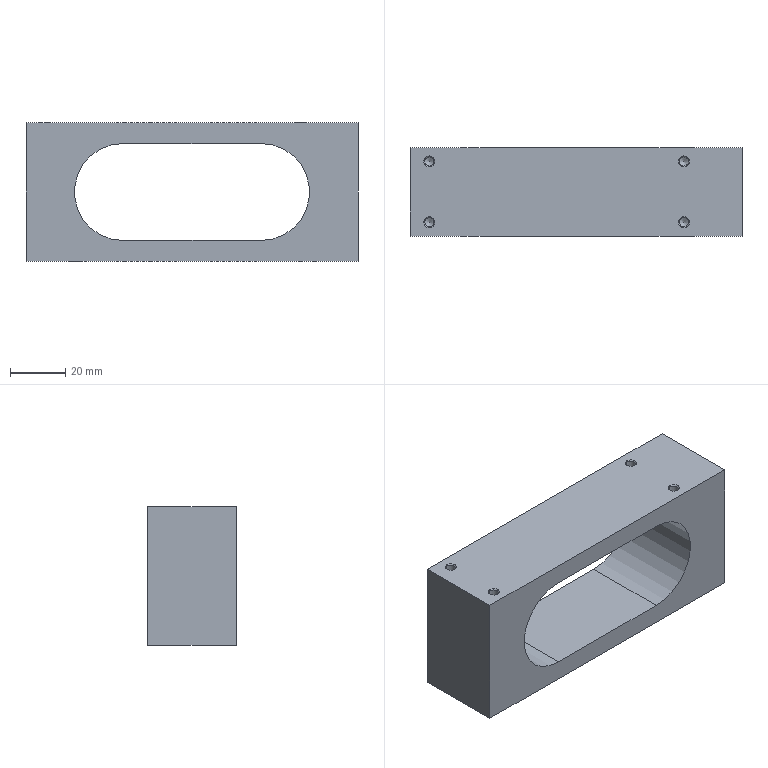Component | NX | SUPPORT_BLOCK_2 | 1 solid | 34 faces | volume 103798 mm3 | cone 16 | cylinder 10 | plane 8 | commonest cylinder face diameters 3.3 x4 5 x4 35 x2